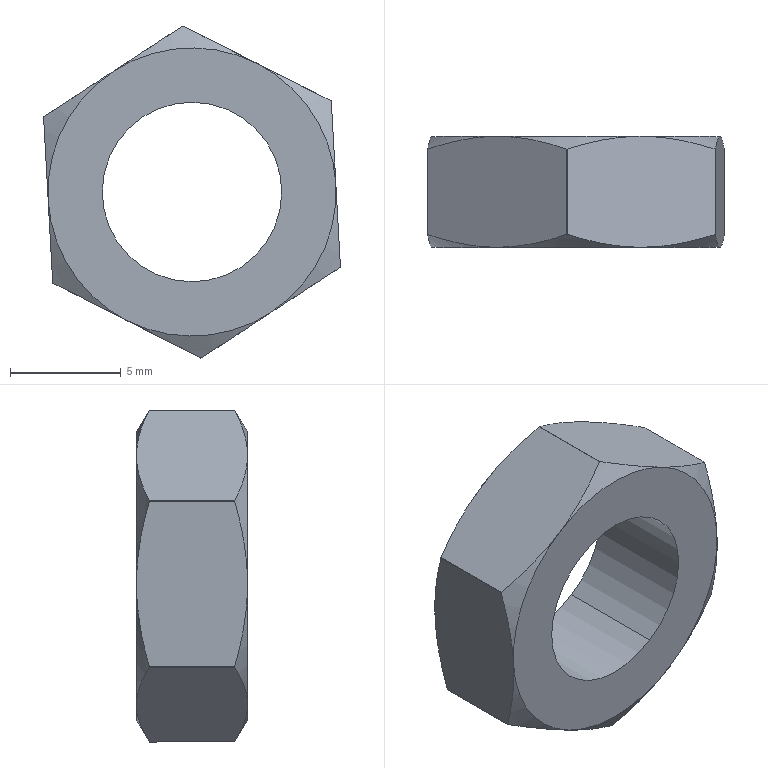Component | SolidWorks | UST8_60-1_NUT_K8-1 | 1 solid | 28 faces | volume 469 mm3 | cone 12 | cylinder 8 | plane 8 | commonest cylinder face diameters 15 x6 8.1 x2